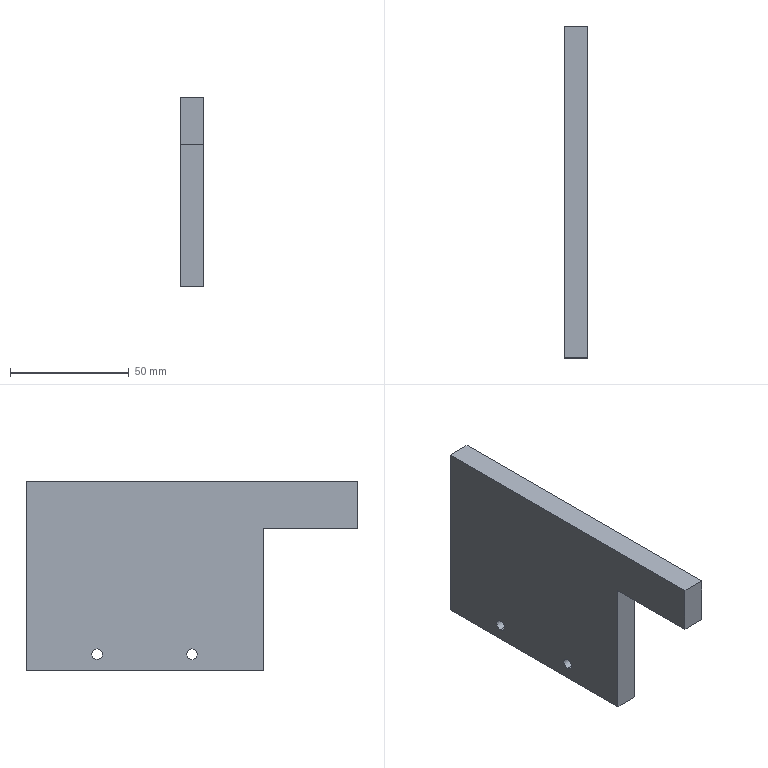Component | SolidWorks | Q1-A12-S21-Q4-06B-9 | 1 solid | 18 faces | box 10 x 140 x 80 mm | volume 87380 mm3 | plane 10 | cylinder 8 | commonest cylinder face diameters 8 x4 4.5 x4 | material White Plastic Steel POM
build123d program:
from build123d import *

# Parameters (mm, degrees)
SKETCH1_W                                       = 80
SKETCH1_H                                       = 140
BOSS_EXTRUDE1_DEPTH                             = 10
SKETCH4_W                                       = 60
SKETCH4_H                                       = 40
CUT_EXTRUDE1_DEPTH                              = 82.24
M4_HEX_SOCKET_HEAD_CAP_SCREW_CBORE1_D           = 4.5
M4_HEX_SOCKET_HEAD_CAP_SCREW_CBORE1_CBORE_D     = 8
M4_HEX_SOCKET_HEAD_CAP_SCREW_CBORE1_CBORE_DEPTH = 4.4


with BuildPart() as part:
    # Sketch1 → Boss-Extrude1 (new body)
    with BuildSketch(Plane.XY):
        Rectangle(SKETCH1_W, SKETCH1_H)
    extrude(amount=BOSS_EXTRUDE1_DEPTH)

    # Sketch4 → Cut-Extrude1 (cut, through all)
    with BuildSketch(Plane.XY.offset(10)):
        with Locations((10, -50)):
            Rectangle(SKETCH4_W, SKETCH4_H)
    extrude(amount=-CUT_EXTRUDE1_DEPTH, mode=Mode.SUBTRACT)

    # M4 Hex Socket Head Cap Screw CBORE1 (through all)
    with Locations(Plane.XY.offset(10)):
        with Locations((33, 40), (33, 0)):
            CounterBoreHole(M4_HEX_SOCKET_HEAD_CAP_SCREW_CBORE1_D / 2, M4_HEX_SOCKET_HEAD_CAP_SCREW_CBORE1_CBORE_D / 2, M4_HEX_SOCKET_HEAD_CAP_SCREW_CBORE1_CBORE_DEPTH)


solid = part.part

# Placed as in the assembly
solid = solid.moved(Location((978.5, 30, 190), (0, 90, 0)))
STEP:
#1=COLOUR_RGB('',0.7922,0.8196,0.9333);
#2=FILL_AREA_STYLE_COLOUR('',#1);
#3=FILL_AREA_STYLE('',(#2));
#4=SURFACE_STYLE_FILL_AREA(#3);
#5=SURFACE_SIDE_STYLE('',(#4));
#6=SURFACE_STYLE_USAGE(.BOTH.,#5);
#7=PRESENTATION_STYLE_ASSIGNMENT((#6));
#8=CARTESIAN_POINT('',(38.744,2.756,6.339));
#9=VERTEX_POINT('',#8);
#10=CARTESIAN_POINT('',(38.744,2.756,6.024));
#11=VERTEX_POINT('',#10);
#12=CARTESIAN_POINT('',(38.744,2.756,6.181));
#13=DIRECTION('',(1.,-0.,-0.));
#14=DIRECTION('',(0.,0.,-1.));
#15=AXIS2_PLACEMENT_3D('',#12,#13,#14);
#16=CIRCLE('',#15,0.1575);
#17=EDGE_CURVE('',#9,#11,#16,.T.);
#18=ORIENTED_EDGE('',*,*,#17,.F.);
#19=CARTESIAN_POINT('',(38.917,2.756,6.339));
#20=VERTEX_POINT('',#19);
#21=CARTESIAN_POINT('',(38.917,2.756,6.339));
#22=DIRECTION('',(1.,-0.,-0.));
#23=VECTOR('',#22,39.37);
#24=LINE('',#21,#23);
#25=EDGE_CURVE('',#9,#20,#24,.T.);
#26=ORIENTED_EDGE('',*,*,#25,.T.);
#27=CARTESIAN_POINT('',(38.917,2.756,6.024));
#28=VERTEX_POINT('',#27);
#29=CARTESIAN_POINT('',(38.917,2.756,6.181));
#30=DIRECTION('',(1.,-0.,-0.));
#31=DIRECTION('',(0.,0.,-1.));
#32=AXIS2_PLACEMENT_3D('',#29,#30,#31);
#33=CIRCLE('',#32,0.1575);
#34=EDGE_CURVE('',#20,#28,#33,.T.);
#35=ORIENTED_EDGE('',*,*,#34,.T.);
#36=CARTESIAN_POINT('',(38.917,2.756,6.024));
#37=DIRECTION('',(1.,-0.,-0.));
#38=VECTOR('',#37,39.37);
#39=LINE('',#36,#38);
#40=EDGE_CURVE('',#11,#28,#39,.T.);
#41=ORIENTED_EDGE('',*,*,#40,.F.);
#42=EDGE_LOOP('',(#18,#26,#35,#41));
#43=FACE_OUTER_BOUND('',#42,.T.);
#44=CARTESIAN_POINT('',(38.917,2.756,6.181));
#45=DIRECTION('',(1.,-0.,-0.));
#46=DIRECTION('',(0.,0.,-1.));
#47=AXIS2_PLACEMENT_3D('',#44,#45,#46);
#48=CYLINDRICAL_SURFACE('',#47,0.1575);
#49=ADVANCED_FACE('',(#43),#48,.F.);
#50=CARTESIAN_POINT('',(38.524,2.756,6.27));
#51=VERTEX_POINT('',#50);
#52=CARTESIAN_POINT('',(38.524,2.756,6.093));
#53=VERTEX_POINT('',#52);
#54=CARTESIAN_POINT('',(38.524,2.756,6.181));
#55=DIRECTION('',(1.,-0.,-0.));
#56=DIRECTION('',(0.,0.,-1.));
#57=AXIS2_PLACEMENT_3D('',#54,#55,#56);
#58=CIRCLE('',#57,0.08858);
#59=EDGE_CURVE('',#51,#53,#58,.T.);
#60=ORIENTED_EDGE('',*,*,#59,.F.);
#61=CARTESIAN_POINT('',(38.744,2.756,6.27));
#62=VERTEX_POINT('',#61);
#63=CARTESIAN_POINT('',(38.917,2.756,6.27));
#64=DIRECTION('',(1.,-0.,-0.));
#65=VECTOR('',#64,39.37);
#66=LINE('',#63,#65);
#67=EDGE_CURVE('',#51,#62,#66,.T.);
#68=ORIENTED_EDGE('',*,*,#67,.T.);
#69=CARTESIAN_POINT('',(38.744,2.756,6.093));
#70=VERTEX_POINT('',#69);
#71=CARTESIAN_POINT('',(38.744,2.756,6.181));
#72=DIRECTION('',(1.,-0.,-0.));
#73=DIRECTION('',(0.,0.,-1.));
#74=AXIS2_PLACEMENT_3D('',#71,#72,#73);
#75=CIRCLE('',#74,0.08858);
#76=EDGE_CURVE('',#62,#70,#75,.T.);
#77=ORIENTED_EDGE('',*,*,#76,.T.);
#78=CARTESIAN_POINT('',(38.917,2.756,6.093));
#79=DIRECTION('',(1.,-0.,-0.));
#80=VECTOR('',#79,39.37);
#81=LINE('',#78,#80);
#82=EDGE_CURVE('',#53,#70,#81,.T.);
#83=ORIENTED_EDGE('',*,*,#82,.F.);
#84=EDGE_LOOP('',(#60,#68,#77,#83));
#85=FACE_OUTER_BOUND('',#84,.T.);
#86=CARTESIAN_POINT('',(38.917,2.756,6.181));
#87=DIRECTION('',(1.,-0.,-0.));
#88=DIRECTION('',(0.,0.,-1.));
#89=AXIS2_PLACEMENT_3D('',#86,#87,#88);
#90=CYLINDRICAL_SURFACE('',#89,0.08858);
#91=ADVANCED_FACE('',(#85),#90,.F.);
#92=CARTESIAN_POINT('',(38.744,1.181,6.339));
#93=VERTEX_POINT('',#92);
#94=CARTESIAN_POINT('',(38.744,1.181,6.024));
#95=VERTEX_POINT('',#94);
#96=CARTESIAN_POINT('',(38.744,1.181,6.181));
#97=DIRECTION('',(1.,-0.,-0.));
#98=DIRECTION('',(0.,0.,-1.));
#99=AXIS2_PLACEMENT_3D('',#96,#97,#98);
#100=CIRCLE('',#99,0.1575);
#101=EDGE_CURVE('',#93,#95,#100,.T.);
#102=ORIENTED_EDGE('',*,*,#101,.F.);
#103=CARTESIAN_POINT('',(38.917,1.181,6.339));
#104=VERTEX_POINT('',#103);
#105=CARTESIAN_POINT('',(38.917,1.181,6.339));
#106=DIRECTION('',(1.,-0.,-0.));
#107=VECTOR('',#106,39.37);
#108=LINE('',#105,#107);
#109=EDGE_CURVE('',#93,#104,#108,.T.);
#110=ORIENTED_EDGE('',*,*,#109,.T.);
#111=CARTESIAN_POINT('',(38.917,1.181,6.024));
#112=VERTEX_POINT('',#111);
#113=CARTESIAN_POINT('',(38.917,1.181,6.181));
#114=DIRECTION('',(1.,-0.,-0.));
#115=DIRECTION('',(0.,0.,-1.));
#116=AXIS2_PLACEMENT_3D('',#113,#114,#115);
#117=CIRCLE('',#116,0.1575);
#118=EDGE_CURVE('',#104,#112,#117,.T.);
#119=ORIENTED_EDGE('',*,*,#118,.T.);
#120=CARTESIAN_POINT('',(38.917,1.181,6.024));
#121=DIRECTION('',(1.,-0.,-0.));
#122=VECTOR('',#121,39.37);
#123=LINE('',#120,#122);
#124=EDGE_CURVE('',#95,#112,#123,.T.);
#125=ORIENTED_EDGE('',*,*,#124,.F.);
#126=EDGE_LOOP('',(#102,#110,#119,#125));
#127=FACE_OUTER_BOUND('',#126,.T.);
#128=CARTESIAN_POINT('',(38.917,1.181,6.181));
#129=DIRECTION('',(1.,-0.,-0.));
#130=DIRECTION('',(0.,0.,-1.));
#131=AXIS2_PLACEMENT_3D('',#128,#129,#130);
#132=CYLINDRICAL_SURFACE('',#131,0.1575);
#133=ADVANCED_FACE('',(#127),#132,.F.);
#134=CARTESIAN_POINT('',(38.524,1.181,6.27));
#135=VERTEX_POINT('',#134);
#136=CARTESIAN_POINT('',(38.524,1.181,6.093));
#137=VERTEX_POINT('',#136);
#138=CARTESIAN_POINT('',(38.524,1.181,6.181));
#139=DIRECTION('',(1.,-0.,-0.));
#140=DIRECTION('',(0.,0.,-1.));
#141=AXIS2_PLACEMENT_3D('',#138,#139,#140);
#142=CIRCLE('',#141,0.08858);
#143=EDGE_CURVE('',#135,#137,#142,.T.);
#144=ORIENTED_EDGE('',*,*,#143,.F.);
#145=CARTESIAN_POINT('',(38.744,1.181,6.27));
#146=VERTEX_POINT('',#145);
#147=CARTESIAN_POINT('',(38.917,1.181,6.27));
#148=DIRECTION('',(1.,-0.,-0.));
#149=VECTOR('',#148,39.37);
#150=LINE('',#147,#149);
#151=EDGE_CURVE('',#135,#146,#150,.T.);
#152=ORIENTED_EDGE('',*,*,#151,.T.);
#153=CARTESIAN_POINT('',(38.744,1.181,6.093));
#154=VERTEX_POINT('',#153);
#155=CARTESIAN_POINT('',(38.744,1.181,6.181));
#156=DIRECTION('',(1.,-0.,-0.));
#157=DIRECTION('',(0.,0.,-1.));
#158=AXIS2_PLACEMENT_3D('',#155,#156,#157);
#159=CIRCLE('',#158,0.08858);
#160=EDGE_CURVE('',#146,#154,#159,.T.);
#161=ORIENTED_EDGE('',*,*,#160,.T.);
#162=CARTESIAN_POINT('',(38.917,1.181,6.093));
#163=DIRECTION('',(1.,-0.,-0.));
#164=VECTOR('',#163,39.37);
#165=LINE('',#162,#164);
#166=EDGE_CURVE('',#137,#154,#165,.T.);
#167=ORIENTED_EDGE('',*,*,#166,.F.);
#168=EDGE_LOOP('',(#144,#152,#161,#167));
#169=FACE_OUTER_BOUND('',#168,.T.);
#170=CARTESIAN_POINT('',(38.917,1.181,6.181));
#171=DIRECTION('',(1.,-0.,-0.));
#172=DIRECTION('',(0.,0.,-1.));
#173=AXIS2_PLACEMENT_3D('',#170,#171,#172);
#174=CYLINDRICAL_SURFACE('',#173,0.08858);
#175=ADVANCED_FACE('',(#169),#174,.F.);
#176=CARTESIAN_POINT('',(38.917,-0.,5.906));
#177=VERTEX_POINT('',#176);
#178=CARTESIAN_POINT('',(38.917,3.937,5.906));
#179=VERTEX_POINT('',#178);
#180=CARTESIAN_POINT('',(38.917,-1.575,5.906));
#181=DIRECTION('',(0.,1.,0.));
#182=VECTOR('',#181,39.37);
#183=LINE('',#180,#182);
#184=EDGE_CURVE('',#177,#179,#183,.T.);
#185=ORIENTED_EDGE('',*,*,#184,.F.);
#186=CARTESIAN_POINT('',(38.524,-0.,5.906));
#187=VERTEX_POINT('',#186);
#188=CARTESIAN_POINT('',(38.524,-0.,5.906));
#189=DIRECTION('',(1.,-0.,-0.));
#190=VECTOR('',#189,39.37);
#191=LINE('',#188,#190);
#192=EDGE_CURVE('',#187,#177,#191,.T.);
#193=ORIENTED_EDGE('',*,*,#192,.F.);
#194=CARTESIAN_POINT('',(38.524,3.937,5.906));
#195=VERTEX_POINT('',#194);
#196=CARTESIAN_POINT('',(38.524,-1.575,5.906));
#197=DIRECTION('',(0.,1.,0.));
#198=VECTOR('',#197,39.37);
#199=LINE('',#196,#198);
#200=EDGE_CURVE('',#187,#195,#199,.T.);
#201=ORIENTED_EDGE('',*,*,#200,.T.);
#202=CARTESIAN_POINT('',(38.917,3.937,5.906));
#203=DIRECTION('',(-1.,0.,0.));
#204=VECTOR('',#203,39.37);
#205=LINE('',#202,#204);
#206=EDGE_CURVE('',#179,#195,#205,.T.);
#207=ORIENTED_EDGE('',*,*,#206,.F.);
#208=EDGE_LOOP('',(#185,#193,#201,#207));
#209=FACE_OUTER_BOUND('',#208,.T.);
#210=CARTESIAN_POINT('',(38.917,-1.575,5.906));
#211=DIRECTION('',(0.,-0.,1.));
#212=DIRECTION('',(1.,-0.,-0.));
#213=AXIS2_PLACEMENT_3D('',#210,#211,#212);
#214=PLANE('',#213);
#215=ADVANCED_FACE('',(#209),#214,.F.);
#216=CARTESIAN_POINT('',(38.524,3.937,9.055));
#217=VERTEX_POINT('',#216);
#218=CARTESIAN_POINT('',(38.524,3.937,9.055));
#219=DIRECTION('',(0.,0.,1.));
#220=VECTOR('',#219,39.37);
#221=LINE('',#218,#220);
#222=EDGE_CURVE('',#195,#217,#221,.T.);
#223=ORIENTED_EDGE('',*,*,#222,.T.);
#224=CARTESIAN_POINT('',(38.917,3.937,9.055));
#225=VERTEX_POINT('',#224);
#226=CARTESIAN_POINT('',(38.917,3.937,9.055));
#227=DIRECTION('',(-1.,0.,0.));
#228=VECTOR('',#227,39.37);
#229=LINE('',#226,#228);
#230=EDGE_CURVE('',#225,#217,#229,.T.);
#231=ORIENTED_EDGE('',*,*,#230,.F.);
#232=CARTESIAN_POINT('',(38.917,3.937,9.055));
#233=DIRECTION('',(0.,0.,1.));
#234=VECTOR('',#233,39.37);
#235=LINE('',#232,#234);
#236=EDGE_CURVE('',#179,#225,#235,.T.);
#237=ORIENTED_EDGE('',*,*,#236,.F.);
#238=ORIENTED_EDGE('',*,*,#206,.T.);
#239=EDGE_LOOP('',(#223,#231,#237,#238));
#240=FACE_OUTER_BOUND('',#239,.T.);
#241=CARTESIAN_POINT('',(38.917,3.937,9.055));
#242=DIRECTION('',(-0.,-1.,0.));
#243=DIRECTION('',(-1.,0.,0.));
#244=AXIS2_PLACEMENT_3D('',#241,#242,#243);
#245=PLANE('',#244);
#246=ADVANCED_FACE('',(#240),#245,.F.);
#247=CARTESIAN_POINT('',(38.524,-1.575,9.055));
#248=VERTEX_POINT('',#247);
#249=CARTESIAN_POINT('',(38.524,-1.575,9.055));
#250=DIRECTION('',(-0.,-1.,0.));
#251=VECTOR('',#250,39.37);
#252=LINE('',#249,#251);
#253=EDGE_CURVE('',#217,#248,#252,.T.);
#254=ORIENTED_EDGE('',*,*,#253,.T.);
#255=CARTESIAN_POINT('',(38.917,-1.575,9.055));
#256=VERTEX_POINT('',#255);
#257=CARTESIAN_POINT('',(38.917,-1.575,9.055));
#258=DIRECTION('',(-1.,0.,0.));
#259=VECTOR('',#258,39.37);
#260=LINE('',#257,#259);
#261=EDGE_CURVE('',#256,#248,#260,.T.);
#262=ORIENTED_EDGE('',*,*,#261,.F.);
#263=CARTESIAN_POINT('',(38.917,-1.575,9.055));
#264=DIRECTION('',(-0.,-1.,0.));
#265=VECTOR('',#264,39.37);
#266=LINE('',#263,#265);
#267=EDGE_CURVE('',#225,#256,#266,.T.);
#268=ORIENTED_EDGE('',*,*,#267,.F.);
#269=ORIENTED_EDGE('',*,*,#230,.T.);
#270=EDGE_LOOP('',(#254,#262,#268,#269));
#271=FACE_OUTER_BOUND('',#270,.T.);
#272=CARTESIAN_POINT('',(38.917,-1.575,9.055));
#273=DIRECTION('',(-0.,0.,-1.));
#274=DIRECTION('',(-1.,0.,0.));
#275=AXIS2_PLACEMENT_3D('',#272,#273,#274);
#276=PLANE('',#275);
#277=ADVANCED_FACE('',(#271),#276,.F.);
#278=CARTESIAN_POINT('',(38.524,-1.575,8.268));
#279=VERTEX_POINT('',#278);
#280=CARTESIAN_POINT('',(38.524,-1.575,9.055));
#281=DIRECTION('',(-0.,0.,-1.));
#282=VECTOR('',#281,39.37);
#283=LINE('',#280,#282);
#284=EDGE_CURVE('',#248,#279,#283,.T.);
#285=ORIENTED_EDGE('',*,*,#284,.T.);
#286=CARTESIAN_POINT('',(38.917,-1.575,8.268));
#287=VERTEX_POINT('',#286);
#288=CARTESIAN_POINT('',(38.524,-1.575,8.268));
#289=DIRECTION('',(1.,-0.,-0.));
#290=VECTOR('',#289,39.37);
#291=LINE('',#288,#290);
#292=EDGE_CURVE('',#279,#287,#291,.T.);
#293=ORIENTED_EDGE('',*,*,#292,.T.);
#294=CARTESIAN_POINT('',(38.917,-1.575,9.055));
#295=DIRECTION('',(-0.,0.,-1.));
#296=VECTOR('',#295,39.37);
#297=LINE('',#294,#296);
#298=EDGE_CURVE('',#256,#287,#297,.T.);
#299=ORIENTED_EDGE('',*,*,#298,.F.);
#300=ORIENTED_EDGE('',*,*,#261,.T.);
#301=EDGE_LOOP('',(#285,#293,#299,#300));
#302=FACE_OUTER_BOUND('',#301,.T.);
#303=CARTESIAN_POINT('',(38.917,-1.575,9.055));
#304=DIRECTION('',(0.,1.,0.));
#305=DIRECTION('',(1.,-0.,-0.));
#306=AXIS2_PLACEMENT_3D('',#303,#304,#305);
#307=PLANE('',#306);
#308=ADVANCED_FACE('',(#302),#307,.F.);
#309=CARTESIAN_POINT('',(38.917,2.756,6.181));
#310=DIRECTION('',(1.,-0.,-0.));
#311=DIRECTION('',(0.,0.,-1.));
#312=AXIS2_PLACEMENT_3D('',#309,#310,#311);
#313=CIRCLE('',#312,0.1575);
#314=EDGE_CURVE('',#28,#20,#313,.T.);
#315=ORIENTED_EDGE('',*,*,#314,.F.);
#316=ORIENTED_EDGE('',*,*,#34,.F.);
#317=EDGE_LOOP('',(#315,#316));
#318=FACE_BOUND('',#317,.T.);
#319=CARTESIAN_POINT('',(38.917,1.181,6.181));
#320=DIRECTION('',(1.,-0.,-0.));
#321=DIRECTION('',(0.,0.,-1.));
#322=AXIS2_PLACEMENT_3D('',#319,#320,#321);
#323=CIRCLE('',#322,0.1575);
#324=EDGE_CURVE('',#112,#104,#323,.T.);
#325=ORIENTED_EDGE('',*,*,#324,.F.);
#326=ORIENTED_EDGE('',*,*,#118,.F.);
#327=EDGE_LOOP('',(#325,#326));
#328=FACE_BOUND('',#327,.T.);
#329=ORIENTED_EDGE('',*,*,#298,.T.);
#330=CARTESIAN_POINT('',(38.917,-0.,8.268));
#331=VERTEX_POINT('',#330);
#332=CARTESIAN_POINT('',(38.917,-1.575,8.268));
#333=DIRECTION('',(-0.,-1.,0.));
#334=VECTOR('',#333,39.37);
#335=LINE('',#332,#334);
#336=EDGE_CURVE('',#331,#287,#335,.T.);
#337=ORIENTED_EDGE('',*,*,#336,.F.);
#338=CARTESIAN_POINT('',(38.917,-0.,5.906));
#339=DIRECTION('',(0.,-0.,1.));
#340=VECTOR('',#339,39.37);
#341=LINE('',#338,#340);
#342=EDGE_CURVE('',#177,#331,#341,.T.);
#343=ORIENTED_EDGE('',*,*,#342,.F.);
#344=ORIENTED_EDGE('',*,*,#184,.T.);
#345=ORIENTED_EDGE('',*,*,#236,.T.);
#346=ORIENTED_EDGE('',*,*,#267,.T.);
#347=EDGE_LOOP('',(#329,#337,#343,#344,#345,#346));
#348=FACE_OUTER_BOUND('',#347,.T.);
#349=CARTESIAN_POINT('',(38.917,1.181,7.48));
#350=DIRECTION('',(-1.,0.,0.));
#351=DIRECTION('',(0.,0.,1.));
#352=AXIS2_PLACEMENT_3D('',#349,#350,#351);
#353=PLANE('',#352);
#354=ADVANCED_FACE('',(#318,#328,#348),#353,.F.);
#355=CARTESIAN_POINT('',(38.524,2.756,6.181));
#356=DIRECTION('',(1.,-0.,-0.));
#357=DIRECTION('',(0.,0.,-1.));
#358=AXIS2_PLACEMENT_3D('',#355,#356,#357);
#359=CIRCLE('',#358,0.08858);
#360=EDGE_CURVE('',#53,#51,#359,.T.);
#361=ORIENTED_EDGE('',*,*,#360,.T.);
#362=ORIENTED_EDGE('',*,*,#59,.T.);
#363=EDGE_LOOP('',(#361,#362));
#364=FACE_BOUND('',#363,.T.);
#365=CARTESIAN_POINT('',(38.524,1.181,6.181));
#366=DIRECTION('',(1.,-0.,-0.));
#367=DIRECTION('',(0.,0.,-1.));
#368=AXIS2_PLACEMENT_3D('',#365,#366,#367);
#369=CIRCLE('',#368,0.08858);
#370=EDGE_CURVE('',#137,#135,#369,.T.);
#371=ORIENTED_EDGE('',*,*,#370,.T.);
#372=ORIENTED_EDGE('',*,*,#143,.T.);
#373=EDGE_LOOP('',(#371,#372));
#374=FACE_BOUND('',#373,.T.);
#375=CARTESIAN_POINT('',(38.524,-0.,8.268));
#376=VERTEX_POINT('',#375);
#377=CARTESIAN_POINT('',(38.524,-1.575,8.268));
#378=DIRECTION('',(-0.,-1.,0.));
#379=VECTOR('',#378,39.37);
#380=LINE('',#377,#379);
#381=EDGE_CURVE('',#376,#279,#380,.T.);
#382=ORIENTED_EDGE('',*,*,#381,.T.);
#383=ORIENTED_EDGE('',*,*,#284,.F.);
#384=ORIENTED_EDGE('',*,*,#253,.F.);
#385=ORIENTED_EDGE('',*,*,#222,.F.);
#386=ORIENTED_EDGE('',*,*,#200,.F.);
#387=CARTESIAN_POINT('',(38.524,-0.,5.906));
#388=DIRECTION('',(0.,-0.,1.));
#389=VECTOR('',#388,39.37);
#390=LINE('',#387,#389);
#391=EDGE_CURVE('',#187,#376,#390,.T.);
#392=ORIENTED_EDGE('',*,*,#391,.T.);
#393=EDGE_LOOP('',(#382,#383,#384,#385,#386,#392));
#394=FACE_OUTER_BOUND('',#393,.T.);
#395=CARTESIAN_POINT('',(38.524,1.181,7.48));
#396=DIRECTION('',(-1.,0.,0.));
#397=DIRECTION('',(0.,0.,1.));
#398=AXIS2_PLACEMENT_3D('',#395,#396,#397);
#399=PLANE('',#398);
#400=ADVANCED_FACE('',(#364,#374,#394),#399,.T.);
#401=ORIENTED_EDGE('',*,*,#336,.T.);
#402=ORIENTED_EDGE('',*,*,#292,.F.);
#403=ORIENTED_EDGE('',*,*,#381,.F.);
#404=CARTESIAN_POINT('',(38.524,-0.,8.268));
#405=DIRECTION('',(1.,-0.,-0.));
#406=VECTOR('',#405,39.37);
#407=LINE('',#404,#406);
#408=EDGE_CURVE('',#376,#331,#407,.T.);
#409=ORIENTED_EDGE('',*,*,#408,.T.);
#410=EDGE_LOOP('',(#401,#402,#403,#409));
#411=FACE_OUTER_BOUND('',#410,.T.);
#412=CARTESIAN_POINT('',(38.524,-1.575,8.268));
#413=DIRECTION('',(0.,-0.,1.));
#414=DIRECTION('',(1.,-0.,-0.));
#415=AXIS2_PLACEMENT_3D('',#412,#413,#414);
#416=PLANE('',#415);
#417=ADVANCED_FACE('',(#411),#416,.F.);
#418=ORIENTED_EDGE('',*,*,#342,.T.);
#419=ORIENTED_EDGE('',*,*,#408,.F.);
#420=ORIENTED_EDGE('',*,*,#391,.F.);
#421=ORIENTED_EDGE('',*,*,#192,.T.);
#422=EDGE_LOOP('',(#418,#419,#420,#421));
#423=FACE_OUTER_BOUND('',#422,.T.);
#424=CARTESIAN_POINT('',(38.524,-0.,5.906));
#425=DIRECTION('',(0.,1.,0.));
#426=DIRECTION('',(0.,-0.,1.));
#427=AXIS2_PLACEMENT_3D('',#424,#425,#426);
#428=PLANE('',#427);
#429=ADVANCED_FACE('',(#423),#428,.F.);
#430=ORIENTED_EDGE('',*,*,#151,.F.);
#431=ORIENTED_EDGE('',*,*,#370,.F.);
#432=ORIENTED_EDGE('',*,*,#166,.T.);
#433=CARTESIAN_POINT('',(38.744,1.181,6.181));
#434=DIRECTION('',(1.,-0.,-0.));
#435=DIRECTION('',(0.,0.,-1.));
#436=AXIS2_PLACEMENT_3D('',#433,#434,#435);
#437=CIRCLE('',#436,0.08858);
#438=EDGE_CURVE('',#154,#146,#437,.T.);
#439=ORIENTED_EDGE('',*,*,#438,.T.);
#440=EDGE_LOOP('',(#430,#431,#432,#439));
#441=FACE_OUTER_BOUND('',#440,.T.);
#442=CARTESIAN_POINT('',(38.917,1.181,6.181));
#443=DIRECTION('',(1.,-0.,-0.));
#444=DIRECTION('',(0.,0.,-1.));
#445=AXIS2_PLACEMENT_3D('',#442,#443,#444);
#446=CYLINDRICAL_SURFACE('',#445,0.08858);
#447=ADVANCED_FACE('',(#441),#446,.F.);
#448=ORIENTED_EDGE('',*,*,#438,.F.);
#449=ORIENTED_EDGE('',*,*,#160,.F.);
#450=EDGE_LOOP('',(#448,#449));
#451=FACE_BOUND('',#450,.T.);
#452=CARTESIAN_POINT('',(38.744,1.181,6.181));
#453=DIRECTION('',(1.,-0.,-0.));
#454=DIRECTION('',(0.,0.,-1.));
#455=AXIS2_PLACEMENT_3D('',#452,#453,#454);
#456=CIRCLE('',#455,0.1575);
#457=EDGE_CURVE('',#95,#93,#456,.T.);
#458=ORIENTED_EDGE('',*,*,#457,.T.);
#459=ORIENTED_EDGE('',*,*,#101,.T.);
#460=EDGE_LOOP('',(#458,#459));
#461=FACE_OUTER_BOUND('',#460,.T.);
#462=CARTESIAN_POINT('',(38.744,1.181,6.093));
#463=DIRECTION('',(-1.,0.,0.));
#464=DIRECTION('',(0.,0.,1.));
#465=AXIS2_PLACEMENT_3D('',#462,#463,#464);
#466=PLANE('',#465);
#467=ADVANCED_FACE('',(#451,#461),#466,.F.);
#468=ORIENTED_EDGE('',*,*,#109,.F.);
#469=ORIENTED_EDGE('',*,*,#457,.F.);
#470=ORIENTED_EDGE('',*,*,#124,.T.);
#471=ORIENTED_EDGE('',*,*,#324,.T.);
#472=EDGE_LOOP('',(#468,#469,#470,#471));
#473=FACE_OUTER_BOUND('',#472,.T.);
#474=CARTESIAN_POINT('',(38.917,1.181,6.181));
#475=DIRECTION('',(1.,-0.,-0.));
#476=DIRECTION('',(0.,0.,-1.));
#477=AXIS2_PLACEMENT_3D('',#474,#475,#476);
#478=CYLINDRICAL_SURFACE('',#477,0.1575);
#479=ADVANCED_FACE('',(#473),#478,.F.);
#480=ORIENTED_EDGE('',*,*,#67,.F.);
#481=ORIENTED_EDGE('',*,*,#360,.F.);
#482=ORIENTED_EDGE('',*,*,#82,.T.);
#483=CARTESIAN_POINT('',(38.744,2.756,6.181));
#484=DIRECTION('',(1.,-0.,-0.));
#485=DIRECTION('',(0.,0.,-1.));
#486=AXIS2_PLACEMENT_3D('',#483,#484,#485);
#487=CIRCLE('',#486,0.08858);
#488=EDGE_CURVE('',#70,#62,#487,.T.);
#489=ORIENTED_EDGE('',*,*,#488,.T.);
#490=EDGE_LOOP('',(#480,#481,#482,#489));
#491=FACE_OUTER_BOUND('',#490,.T.);
#492=CARTESIAN_POINT('',(38.917,2.756,6.181));
#493=DIRECTION('',(1.,-0.,-0.));
#494=DIRECTION('',(0.,0.,-1.));
#495=AXIS2_PLACEMENT_3D('',#492,#493,#494);
#496=CYLINDRICAL_SURFACE('',#495,0.08858);
#497=ADVANCED_FACE('',(#491),#496,.F.);
#498=ORIENTED_EDGE('',*,*,#488,.F.);
#499=ORIENTED_EDGE('',*,*,#76,.F.);
#500=EDGE_LOOP('',(#498,#499));
#501=FACE_BOUND('',#500,.T.);
#502=CARTESIAN_POINT('',(38.744,2.756,6.181));
#503=DIRECTION('',(1.,-0.,-0.));
#504=DIRECTION('',(0.,0.,-1.));
#505=AXIS2_PLACEMENT_3D('',#502,#503,#504);
#506=CIRCLE('',#505,0.1575);
#507=EDGE_CURVE('',#11,#9,#506,.T.);
#508=ORIENTED_EDGE('',*,*,#507,.T.);
#509=ORIENTED_EDGE('',*,*,#17,.T.);
#510=EDGE_LOOP('',(#508,#509));
#511=FACE_OUTER_BOUND('',#510,.T.);
#512=CARTESIAN_POINT('',(38.744,2.756,6.093));
#513=DIRECTION('',(-1.,0.,0.));
#514=DIRECTION('',(0.,0.,1.));
#515=AXIS2_PLACEMENT_3D('',#512,#513,#514);
#516=PLANE('',#515);
#517=ADVANCED_FACE('',(#501,#511),#516,.F.);
#518=ORIENTED_EDGE('',*,*,#25,.F.);
#519=ORIENTED_EDGE('',*,*,#507,.F.);
#520=ORIENTED_EDGE('',*,*,#40,.T.);
#521=ORIENTED_EDGE('',*,*,#314,.T.);
#522=EDGE_LOOP('',(#518,#519,#520,#521));
#523=FACE_OUTER_BOUND('',#522,.T.);
#524=CARTESIAN_POINT('',(38.917,2.756,6.181));
#525=DIRECTION('',(1.,-0.,-0.));
#526=DIRECTION('',(0.,0.,-1.));
#527=AXIS2_PLACEMENT_3D('',#524,#525,#526);
#528=CYLINDRICAL_SURFACE('',#527,0.1575);
#529=ADVANCED_FACE('',(#523),#528,.F.);
#530=CLOSED_SHELL('',(#49,#91,#133,#175,#215,#246,#277,#308,#354,#400,#417,#429,#447,#467,#479,#497,#517,#529));
#531=MANIFOLD_SOLID_BREP('',#530);
#532=STYLED_ITEM('',(#7),#531);
#533=(LENGTH_UNIT()NAMED_UNIT(*)SI_UNIT($,.METRE.));
#534=LENGTH_MEASURE_WITH_UNIT(LENGTH_MEASURE(0.0254),#533);
#535=DIMENSIONAL_EXPONENTS(1.,0.,0.,0.,0.,0.,0.);
#536=(CONVERSION_BASED_UNIT('',#534)LENGTH_UNIT()NAMED_UNIT(#535));
#537=UNCERTAINTY_MEASURE_WITH_UNIT(LENGTH_MEASURE(0.00001),#536,'','');
#538=(NAMED_UNIT(*)PLANE_ANGLE_UNIT()SI_UNIT($,.RADIAN.));
#539=(NAMED_UNIT(*)SI_UNIT($,.STERADIAN.)SOLID_ANGLE_UNIT());
#540=(GEOMETRIC_REPRESENTATION_CONTEXT(3)GLOBAL_UNCERTAINTY_ASSIGNED_CONTEXT((#537))GLOBAL_UNIT_ASSIGNED_CONTEXT((#536,#538,#539))REPRESENTATION_CONTEXT('',''));
#541=MECHANICAL_DESIGN_GEOMETRIC_PRESENTATION_REPRESENTATION('',(#532),#540);
#542=CARTESIAN_POINT('',(0.,0.,0.));
#543=DIRECTION('',(0.,0.,1.));
#544=DIRECTION('',(1.,0.,0.));
#545=AXIS2_PLACEMENT_3D('',#542,#543,#544);
#546=(LENGTH_UNIT()NAMED_UNIT(*)SI_UNIT($,.METRE.));
#547=LENGTH_MEASURE_WITH_UNIT(LENGTH_MEASURE(0.0254),#546);
#548=DIMENSIONAL_EXPONENTS(1.,0.,0.,0.,0.,0.,0.);
#549=(CONVERSION_BASED_UNIT('',#547)LENGTH_UNIT()NAMED_UNIT(#548));
#550=UNCERTAINTY_MEASURE_WITH_UNIT(LENGTH_MEASURE(0.00001),#549,'','');
#551=(NAMED_UNIT(*)PLANE_ANGLE_UNIT()SI_UNIT($,.RADIAN.));
#552=(NAMED_UNIT(*)SI_UNIT($,.STERADIAN.)SOLID_ANGLE_UNIT());
#553=(GEOMETRIC_REPRESENTATION_CONTEXT(3)GLOBAL_UNCERTAINTY_ASSIGNED_CONTEXT((#550))GLOBAL_UNIT_ASSIGNED_CONTEXT((#549,#551,#552))REPRESENTATION_CONTEXT('',''));
#554=ADVANCED_BREP_SHAPE_REPRESENTATION('',(#531,#545),#553);
#555=PRESENTATION_LAYER_ASSIGNMENT('','',(#532));